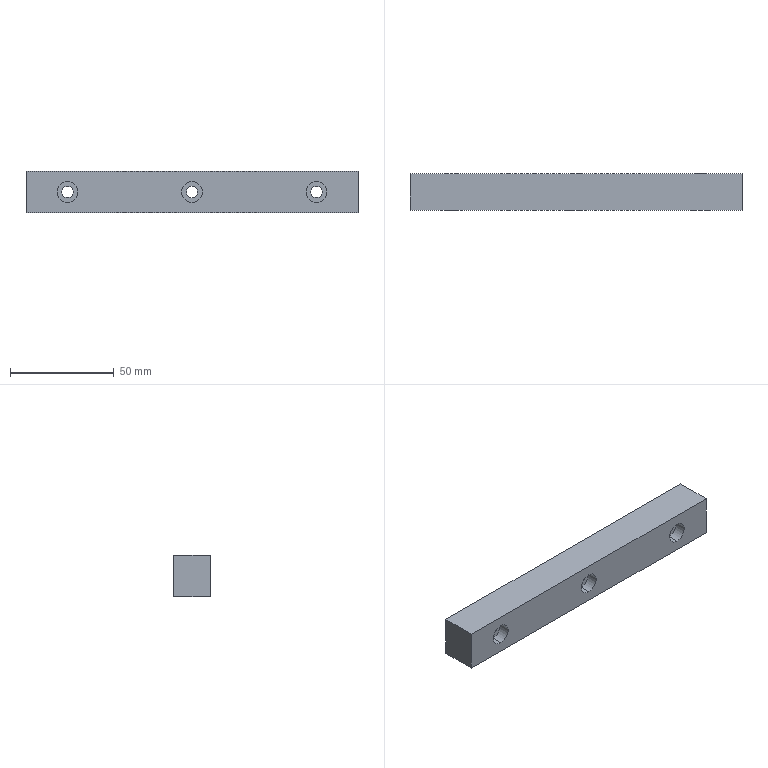Component | SolidWorks | GuideRailHIWINHGH20CA1R220-Z0-C-1 | 1 solid | 21 faces | box 160 x 17.5 x 20 mm | volume 53865 mm3 | cylinder 12 | plane 9 | commonest cylinder face diameters 5.5 x6 10 x6
build123d program:
from build123d import *

# Parameters (mm, degrees)
SKETCH1_W                                           = 160
SKETCH1_H                                           = 20
EXTRUDE1_DEPTH                                      = 17.5
CBORE_FOR_M5_HEX_SOCKET_HEAD_CAP_SCREW1_D           = 5.5
CBORE_FOR_M5_HEX_SOCKET_HEAD_CAP_SCREW1_CBORE_D     = 10
CBORE_FOR_M5_HEX_SOCKET_HEAD_CAP_SCREW1_CBORE_DEPTH = 5.4
LPATTERN1_COUNT                                     = 3
LPATTERN1_PITCH                                     = 60


with BuildPart() as part:
    # Sketch1 → Extrude1 (new body)
    with BuildSketch(Plane(origin=(0, 0, 0), x_dir=(1, 0, 0), z_dir=(0, 1, 0))):
        Rectangle(SKETCH1_W, SKETCH1_H)
    extrude(amount=EXTRUDE1_DEPTH)

    # CBORE for M5 Hex Socket Head Cap Screw1 (through all)
    with Locations(Plane(origin=(0, 17.5, 0), x_dir=(-1, 0, 0), z_dir=(0, 1, 0))):
        with Locations((-60, 0)):
            cbore_for_m5_hex_socket_head_cap_screw1 = CounterBoreHole(CBORE_FOR_M5_HEX_SOCKET_HEAD_CAP_SCREW1_D / 2, CBORE_FOR_M5_HEX_SOCKET_HEAD_CAP_SCREW1_CBORE_D / 2, CBORE_FOR_M5_HEX_SOCKET_HEAD_CAP_SCREW1_CBORE_DEPTH)

    # LPattern1: CBORE for M5 Hex Socket Head Cap Screw1 ×3
    with Locations(*[(-i * LPATTERN1_PITCH, 0, 0) for i in range(1, LPATTERN1_COUNT)]):
        add(cbore_for_m5_hex_socket_head_cap_screw1, mode=Mode.SUBTRACT)


solid = part.part

# Placed as in the assembly
solid = solid.moved(Location((-41.5, -10, -55), (180, 0, 0)))
STEP:
#1=COLOUR_RGB('',0.7922,0.8196,0.9333);
#2=FILL_AREA_STYLE_COLOUR('',#1);
#3=FILL_AREA_STYLE('',(#2));
#4=SURFACE_STYLE_FILL_AREA(#3);
#5=SURFACE_SIDE_STYLE('',(#4));
#6=SURFACE_STYLE_USAGE(.BOTH.,#5);
#7=PRESENTATION_STYLE_ASSIGNMENT((#6));
#8=CARTESIAN_POINT('',(0.7283,-0.3937,-2.274));
#9=VERTEX_POINT('',#8);
#10=CARTESIAN_POINT('',(0.7283,-0.3937,-2.057));
#11=VERTEX_POINT('',#10);
#12=CARTESIAN_POINT('',(0.7283,-0.3937,-2.165));
#13=DIRECTION('',(-0.,-1.,0.));
#14=DIRECTION('',(0.,0.,1.));
#15=AXIS2_PLACEMENT_3D('',#12,#13,#14);
#16=CIRCLE('',#15,0.1083);
#17=EDGE_CURVE('',#9,#11,#16,.T.);
#18=ORIENTED_EDGE('',*,*,#17,.F.);
#19=CARTESIAN_POINT('',(0.7283,-0.8701,-2.274));
#20=VERTEX_POINT('',#19);
#21=CARTESIAN_POINT('',(0.7283,-1.083,-2.274));
#22=DIRECTION('',(-0.,-1.,0.));
#23=VECTOR('',#22,39.37);
#24=LINE('',#21,#23);
#25=EDGE_CURVE('',#9,#20,#24,.T.);
#26=ORIENTED_EDGE('',*,*,#25,.T.);
#27=CARTESIAN_POINT('',(0.7283,-0.8701,-2.057));
#28=VERTEX_POINT('',#27);
#29=CARTESIAN_POINT('',(0.7283,-0.8701,-2.165));
#30=DIRECTION('',(-0.,-1.,0.));
#31=DIRECTION('',(0.,0.,1.));
#32=AXIS2_PLACEMENT_3D('',#29,#30,#31);
#33=CIRCLE('',#32,0.1083);
#34=EDGE_CURVE('',#20,#28,#33,.T.);
#35=ORIENTED_EDGE('',*,*,#34,.T.);
#36=CARTESIAN_POINT('',(0.7283,-1.083,-2.057));
#37=DIRECTION('',(-0.,-1.,0.));
#38=VECTOR('',#37,39.37);
#39=LINE('',#36,#38);
#40=EDGE_CURVE('',#11,#28,#39,.T.);
#41=ORIENTED_EDGE('',*,*,#40,.F.);
#42=EDGE_LOOP('',(#18,#26,#35,#41));
#43=FACE_OUTER_BOUND('',#42,.T.);
#44=CARTESIAN_POINT('',(0.7283,-1.083,-2.165));
#45=DIRECTION('',(-0.,-1.,0.));
#46=DIRECTION('',(0.,0.,1.));
#47=AXIS2_PLACEMENT_3D('',#44,#45,#46);
#48=CYLINDRICAL_SURFACE('',#47,0.1083);
#49=ADVANCED_FACE('',(#43),#48,.F.);
#50=CARTESIAN_POINT('',(0.7283,-0.8701,-2.362));
#51=VERTEX_POINT('',#50);
#52=CARTESIAN_POINT('',(0.7283,-0.8701,-1.969));
#53=VERTEX_POINT('',#52);
#54=CARTESIAN_POINT('',(0.7283,-0.8701,-2.165));
#55=DIRECTION('',(-0.,-1.,0.));
#56=DIRECTION('',(0.,0.,1.));
#57=AXIS2_PLACEMENT_3D('',#54,#55,#56);
#58=CIRCLE('',#57,0.1969);
#59=EDGE_CURVE('',#51,#53,#58,.T.);
#60=ORIENTED_EDGE('',*,*,#59,.F.);
#61=CARTESIAN_POINT('',(0.7283,-1.083,-2.362));
#62=VERTEX_POINT('',#61);
#63=CARTESIAN_POINT('',(0.7283,-1.083,-2.362));
#64=DIRECTION('',(-0.,-1.,0.));
#65=VECTOR('',#64,39.37);
#66=LINE('',#63,#65);
#67=EDGE_CURVE('',#51,#62,#66,.T.);
#68=ORIENTED_EDGE('',*,*,#67,.T.);
#69=CARTESIAN_POINT('',(0.7283,-1.083,-1.969));
#70=VERTEX_POINT('',#69);
#71=CARTESIAN_POINT('',(0.7283,-1.083,-2.165));
#72=DIRECTION('',(-0.,-1.,0.));
#73=DIRECTION('',(0.,0.,1.));
#74=AXIS2_PLACEMENT_3D('',#71,#72,#73);
#75=CIRCLE('',#74,0.1969);
#76=EDGE_CURVE('',#62,#70,#75,.T.);
#77=ORIENTED_EDGE('',*,*,#76,.T.);
#78=CARTESIAN_POINT('',(0.7283,-1.083,-1.969));
#79=DIRECTION('',(-0.,-1.,0.));
#80=VECTOR('',#79,39.37);
#81=LINE('',#78,#80);
#82=EDGE_CURVE('',#53,#70,#81,.T.);
#83=ORIENTED_EDGE('',*,*,#82,.F.);
#84=EDGE_LOOP('',(#60,#68,#77,#83));
#85=FACE_OUTER_BOUND('',#84,.T.);
#86=CARTESIAN_POINT('',(0.7283,-1.083,-2.165));
#87=DIRECTION('',(-0.,-1.,0.));
#88=DIRECTION('',(0.,0.,1.));
#89=AXIS2_PLACEMENT_3D('',#86,#87,#88);
#90=CYLINDRICAL_SURFACE('',#89,0.1969);
#91=ADVANCED_FACE('',(#85),#90,.F.);
#92=CARTESIAN_POINT('',(-1.634,-0.8701,-2.362));
#93=VERTEX_POINT('',#92);
#94=CARTESIAN_POINT('',(-1.634,-0.8701,-1.969));
#95=VERTEX_POINT('',#94);
#96=CARTESIAN_POINT('',(-1.634,-0.8701,-2.165));
#97=DIRECTION('',(-0.,-1.,0.));
#98=DIRECTION('',(0.,0.,1.));
#99=AXIS2_PLACEMENT_3D('',#96,#97,#98);
#100=CIRCLE('',#99,0.1969);
#101=EDGE_CURVE('',#93,#95,#100,.T.);
#102=ORIENTED_EDGE('',*,*,#101,.F.);
#103=CARTESIAN_POINT('',(-1.634,-1.083,-2.362));
#104=VERTEX_POINT('',#103);
#105=CARTESIAN_POINT('',(-1.634,-1.083,-2.362));
#106=DIRECTION('',(-0.,-1.,0.));
#107=VECTOR('',#106,39.37);
#108=LINE('',#105,#107);
#109=EDGE_CURVE('',#93,#104,#108,.T.);
#110=ORIENTED_EDGE('',*,*,#109,.T.);
#111=CARTESIAN_POINT('',(-1.634,-1.083,-1.969));
#112=VERTEX_POINT('',#111);
#113=CARTESIAN_POINT('',(-1.634,-1.083,-2.165));
#114=DIRECTION('',(-0.,-1.,0.));
#115=DIRECTION('',(0.,0.,1.));
#116=AXIS2_PLACEMENT_3D('',#113,#114,#115);
#117=CIRCLE('',#116,0.1969);
#118=EDGE_CURVE('',#104,#112,#117,.T.);
#119=ORIENTED_EDGE('',*,*,#118,.T.);
#120=CARTESIAN_POINT('',(-1.634,-1.083,-1.969));
#121=DIRECTION('',(-0.,-1.,0.));
#122=VECTOR('',#121,39.37);
#123=LINE('',#120,#122);
#124=EDGE_CURVE('',#95,#112,#123,.T.);
#125=ORIENTED_EDGE('',*,*,#124,.F.);
#126=EDGE_LOOP('',(#102,#110,#119,#125));
#127=FACE_OUTER_BOUND('',#126,.T.);
#128=CARTESIAN_POINT('',(-1.634,-1.083,-2.165));
#129=DIRECTION('',(-0.,-1.,0.));
#130=DIRECTION('',(0.,0.,1.));
#131=AXIS2_PLACEMENT_3D('',#128,#129,#130);
#132=CYLINDRICAL_SURFACE('',#131,0.1969);
#133=ADVANCED_FACE('',(#127),#132,.F.);
#134=CARTESIAN_POINT('',(-1.634,-0.3937,-2.274));
#135=VERTEX_POINT('',#134);
#136=CARTESIAN_POINT('',(-1.634,-0.3937,-2.057));
#137=VERTEX_POINT('',#136);
#138=CARTESIAN_POINT('',(-1.634,-0.3937,-2.165));
#139=DIRECTION('',(-0.,-1.,0.));
#140=DIRECTION('',(0.,0.,1.));
#141=AXIS2_PLACEMENT_3D('',#138,#139,#140);
#142=CIRCLE('',#141,0.1083);
#143=EDGE_CURVE('',#135,#137,#142,.T.);
#144=ORIENTED_EDGE('',*,*,#143,.F.);
#145=CARTESIAN_POINT('',(-1.634,-0.8701,-2.274));
#146=VERTEX_POINT('',#145);
#147=CARTESIAN_POINT('',(-1.634,-1.083,-2.274));
#148=DIRECTION('',(-0.,-1.,0.));
#149=VECTOR('',#148,39.37);
#150=LINE('',#147,#149);
#151=EDGE_CURVE('',#135,#146,#150,.T.);
#152=ORIENTED_EDGE('',*,*,#151,.T.);
#153=CARTESIAN_POINT('',(-1.634,-0.8701,-2.057));
#154=VERTEX_POINT('',#153);
#155=CARTESIAN_POINT('',(-1.634,-0.8701,-2.165));
#156=DIRECTION('',(-0.,-1.,0.));
#157=DIRECTION('',(0.,0.,1.));
#158=AXIS2_PLACEMENT_3D('',#155,#156,#157);
#159=CIRCLE('',#158,0.1083);
#160=EDGE_CURVE('',#146,#154,#159,.T.);
#161=ORIENTED_EDGE('',*,*,#160,.T.);
#162=CARTESIAN_POINT('',(-1.634,-1.083,-2.057));
#163=DIRECTION('',(-0.,-1.,0.));
#164=VECTOR('',#163,39.37);
#165=LINE('',#162,#164);
#166=EDGE_CURVE('',#137,#154,#165,.T.);
#167=ORIENTED_EDGE('',*,*,#166,.F.);
#168=EDGE_LOOP('',(#144,#152,#161,#167));
#169=FACE_OUTER_BOUND('',#168,.T.);
#170=CARTESIAN_POINT('',(-1.634,-1.083,-2.165));
#171=DIRECTION('',(-0.,-1.,0.));
#172=DIRECTION('',(0.,0.,1.));
#173=AXIS2_PLACEMENT_3D('',#170,#171,#172);
#174=CYLINDRICAL_SURFACE('',#173,0.1083);
#175=ADVANCED_FACE('',(#169),#174,.F.);
#176=CARTESIAN_POINT('',(-3.996,-0.8701,-2.362));
#177=VERTEX_POINT('',#176);
#178=CARTESIAN_POINT('',(-3.996,-0.8701,-1.969));
#179=VERTEX_POINT('',#178);
#180=CARTESIAN_POINT('',(-3.996,-0.8701,-2.165));
#181=DIRECTION('',(-0.,-1.,0.));
#182=DIRECTION('',(0.,0.,1.));
#183=AXIS2_PLACEMENT_3D('',#180,#181,#182);
#184=CIRCLE('',#183,0.1969);
#185=EDGE_CURVE('',#177,#179,#184,.T.);
#186=ORIENTED_EDGE('',*,*,#185,.F.);
#187=CARTESIAN_POINT('',(-3.996,-1.083,-2.362));
#188=VERTEX_POINT('',#187);
#189=CARTESIAN_POINT('',(-3.996,-1.083,-2.362));
#190=DIRECTION('',(-0.,-1.,0.));
#191=VECTOR('',#190,39.37);
#192=LINE('',#189,#191);
#193=EDGE_CURVE('',#177,#188,#192,.T.);
#194=ORIENTED_EDGE('',*,*,#193,.T.);
#195=CARTESIAN_POINT('',(-3.996,-1.083,-1.969));
#196=VERTEX_POINT('',#195);
#197=CARTESIAN_POINT('',(-3.996,-1.083,-2.165));
#198=DIRECTION('',(-0.,-1.,0.));
#199=DIRECTION('',(0.,0.,1.));
#200=AXIS2_PLACEMENT_3D('',#197,#198,#199);
#201=CIRCLE('',#200,0.1969);
#202=EDGE_CURVE('',#188,#196,#201,.T.);
#203=ORIENTED_EDGE('',*,*,#202,.T.);
#204=CARTESIAN_POINT('',(-3.996,-1.083,-1.969));
#205=DIRECTION('',(-0.,-1.,0.));
#206=VECTOR('',#205,39.37);
#207=LINE('',#204,#206);
#208=EDGE_CURVE('',#179,#196,#207,.T.);
#209=ORIENTED_EDGE('',*,*,#208,.F.);
#210=EDGE_LOOP('',(#186,#194,#203,#209));
#211=FACE_OUTER_BOUND('',#210,.T.);
#212=CARTESIAN_POINT('',(-3.996,-1.083,-2.165));
#213=DIRECTION('',(-0.,-1.,0.));
#214=DIRECTION('',(0.,0.,1.));
#215=AXIS2_PLACEMENT_3D('',#212,#213,#214);
#216=CYLINDRICAL_SURFACE('',#215,0.1969);
#217=ADVANCED_FACE('',(#211),#216,.F.);
#218=CARTESIAN_POINT('',(-3.996,-0.3937,-2.274));
#219=VERTEX_POINT('',#218);
#220=CARTESIAN_POINT('',(-3.996,-0.3937,-2.057));
#221=VERTEX_POINT('',#220);
#222=CARTESIAN_POINT('',(-3.996,-0.3937,-2.165));
#223=DIRECTION('',(-0.,-1.,0.));
#224=DIRECTION('',(0.,0.,1.));
#225=AXIS2_PLACEMENT_3D('',#222,#223,#224);
#226=CIRCLE('',#225,0.1083);
#227=EDGE_CURVE('',#219,#221,#226,.T.);
#228=ORIENTED_EDGE('',*,*,#227,.F.);
#229=CARTESIAN_POINT('',(-3.996,-0.8701,-2.274));
#230=VERTEX_POINT('',#229);
#231=CARTESIAN_POINT('',(-3.996,-1.083,-2.274));
#232=DIRECTION('',(-0.,-1.,0.));
#233=VECTOR('',#232,39.37);
#234=LINE('',#231,#233);
#235=EDGE_CURVE('',#219,#230,#234,.T.);
#236=ORIENTED_EDGE('',*,*,#235,.T.);
#237=CARTESIAN_POINT('',(-3.996,-0.8701,-2.057));
#238=VERTEX_POINT('',#237);
#239=CARTESIAN_POINT('',(-3.996,-0.8701,-2.165));
#240=DIRECTION('',(-0.,-1.,0.));
#241=DIRECTION('',(0.,0.,1.));
#242=AXIS2_PLACEMENT_3D('',#239,#240,#241);
#243=CIRCLE('',#242,0.1083);
#244=EDGE_CURVE('',#230,#238,#243,.T.);
#245=ORIENTED_EDGE('',*,*,#244,.T.);
#246=CARTESIAN_POINT('',(-3.996,-1.083,-2.057));
#247=DIRECTION('',(-0.,-1.,0.));
#248=VECTOR('',#247,39.37);
#249=LINE('',#246,#248);
#250=EDGE_CURVE('',#221,#238,#249,.T.);
#251=ORIENTED_EDGE('',*,*,#250,.F.);
#252=EDGE_LOOP('',(#228,#236,#245,#251));
#253=FACE_OUTER_BOUND('',#252,.T.);
#254=CARTESIAN_POINT('',(-3.996,-1.083,-2.165));
#255=DIRECTION('',(-0.,-1.,0.));
#256=DIRECTION('',(0.,0.,1.));
#257=AXIS2_PLACEMENT_3D('',#254,#255,#256);
#258=CYLINDRICAL_SURFACE('',#257,0.1083);
#259=ADVANCED_FACE('',(#253),#258,.F.);
#260=CARTESIAN_POINT('',(1.516,-0.3937,-2.559));
#261=VERTEX_POINT('',#260);
#262=CARTESIAN_POINT('',(1.516,-0.3937,-1.772));
#263=VERTEX_POINT('',#262);
#264=CARTESIAN_POINT('',(1.516,-0.3937,-2.559));
#265=DIRECTION('',(-0.,0.,1.));
#266=VECTOR('',#265,39.37);
#267=LINE('',#264,#266);
#268=EDGE_CURVE('',#261,#263,#267,.T.);
#269=ORIENTED_EDGE('',*,*,#268,.T.);
#270=CARTESIAN_POINT('',(1.516,-1.083,-1.772));
#271=VERTEX_POINT('',#270);
#272=CARTESIAN_POINT('',(1.516,-1.083,-1.772));
#273=DIRECTION('',(0.,1.,-0.));
#274=VECTOR('',#273,39.37);
#275=LINE('',#272,#274);
#276=EDGE_CURVE('',#271,#263,#275,.T.);
#277=ORIENTED_EDGE('',*,*,#276,.F.);
#278=CARTESIAN_POINT('',(1.516,-1.083,-2.559));
#279=VERTEX_POINT('',#278);
#280=CARTESIAN_POINT('',(1.516,-1.083,-2.559));
#281=DIRECTION('',(-0.,0.,1.));
#282=VECTOR('',#281,39.37);
#283=LINE('',#280,#282);
#284=EDGE_CURVE('',#279,#271,#283,.T.);
#285=ORIENTED_EDGE('',*,*,#284,.F.);
#286=CARTESIAN_POINT('',(1.516,-1.083,-2.559));
#287=DIRECTION('',(0.,1.,-0.));
#288=VECTOR('',#287,39.37);
#289=LINE('',#286,#288);
#290=EDGE_CURVE('',#279,#261,#289,.T.);
#291=ORIENTED_EDGE('',*,*,#290,.T.);
#292=EDGE_LOOP('',(#269,#277,#285,#291));
#293=FACE_OUTER_BOUND('',#292,.T.);
#294=CARTESIAN_POINT('',(1.516,-1.083,-2.559));
#295=DIRECTION('',(-1.,0.,-0.));
#296=DIRECTION('',(0.,-0.,-1.));
#297=AXIS2_PLACEMENT_3D('',#294,#295,#296);
#298=PLANE('',#297);
#299=ADVANCED_FACE('',(#293),#298,.F.);
#300=CARTESIAN_POINT('',(-4.783,-0.3937,-1.772));
#301=VERTEX_POINT('',#300);
#302=CARTESIAN_POINT('',(1.516,-0.3937,-1.772));
#303=DIRECTION('',(-1.,0.,-0.));
#304=VECTOR('',#303,39.37);
#305=LINE('',#302,#304);
#306=EDGE_CURVE('',#263,#301,#305,.T.);
#307=ORIENTED_EDGE('',*,*,#306,.T.);
#308=CARTESIAN_POINT('',(-4.783,-1.083,-1.772));
#309=VERTEX_POINT('',#308);
#310=CARTESIAN_POINT('',(-4.783,-1.083,-1.772));
#311=DIRECTION('',(0.,1.,-0.));
#312=VECTOR('',#311,39.37);
#313=LINE('',#310,#312);
#314=EDGE_CURVE('',#309,#301,#313,.T.);
#315=ORIENTED_EDGE('',*,*,#314,.F.);
#316=CARTESIAN_POINT('',(1.516,-1.083,-1.772));
#317=DIRECTION('',(-1.,0.,-0.));
#318=VECTOR('',#317,39.37);
#319=LINE('',#316,#318);
#320=EDGE_CURVE('',#271,#309,#319,.T.);
#321=ORIENTED_EDGE('',*,*,#320,.F.);
#322=ORIENTED_EDGE('',*,*,#276,.T.);
#323=EDGE_LOOP('',(#307,#315,#321,#322));
#324=FACE_OUTER_BOUND('',#323,.T.);
#325=CARTESIAN_POINT('',(1.516,-1.083,-1.772));
#326=DIRECTION('',(0.,-0.,-1.));
#327=DIRECTION('',(1.,-0.,0.));
#328=AXIS2_PLACEMENT_3D('',#325,#326,#327);
#329=PLANE('',#328);
#330=ADVANCED_FACE('',(#324),#329,.F.);
#331=CARTESIAN_POINT('',(-4.783,-0.3937,-2.559));
#332=VERTEX_POINT('',#331);
#333=CARTESIAN_POINT('',(-4.783,-0.3937,-2.559));
#334=DIRECTION('',(0.,-0.,-1.));
#335=VECTOR('',#334,39.37);
#336=LINE('',#333,#335);
#337=EDGE_CURVE('',#301,#332,#336,.T.);
#338=ORIENTED_EDGE('',*,*,#337,.T.);
#339=CARTESIAN_POINT('',(-4.783,-1.083,-2.559));
#340=VERTEX_POINT('',#339);
#341=CARTESIAN_POINT('',(-4.783,-1.083,-2.559));
#342=DIRECTION('',(0.,1.,-0.));
#343=VECTOR('',#342,39.37);
#344=LINE('',#341,#343);
#345=EDGE_CURVE('',#340,#332,#344,.T.);
#346=ORIENTED_EDGE('',*,*,#345,.F.);
#347=CARTESIAN_POINT('',(-4.783,-1.083,-2.559));
#348=DIRECTION('',(0.,-0.,-1.));
#349=VECTOR('',#348,39.37);
#350=LINE('',#347,#349);
#351=EDGE_CURVE('',#309,#340,#350,.T.);
#352=ORIENTED_EDGE('',*,*,#351,.F.);
#353=ORIENTED_EDGE('',*,*,#314,.T.);
#354=EDGE_LOOP('',(#338,#346,#352,#353));
#355=FACE_OUTER_BOUND('',#354,.T.);
#356=CARTESIAN_POINT('',(-4.783,-1.083,-2.559));
#357=DIRECTION('',(1.,-0.,0.));
#358=DIRECTION('',(-0.,0.,1.));
#359=AXIS2_PLACEMENT_3D('',#356,#357,#358);
#360=PLANE('',#359);
#361=ADVANCED_FACE('',(#355),#360,.F.);
#362=CARTESIAN_POINT('',(1.516,-0.3937,-2.559));
#363=DIRECTION('',(1.,-0.,0.));
#364=VECTOR('',#363,39.37);
#365=LINE('',#362,#364);
#366=EDGE_CURVE('',#332,#261,#365,.T.);
#367=ORIENTED_EDGE('',*,*,#366,.T.);
#368=ORIENTED_EDGE('',*,*,#290,.F.);
#369=CARTESIAN_POINT('',(1.516,-1.083,-2.559));
#370=DIRECTION('',(1.,-0.,0.));
#371=VECTOR('',#370,39.37);
#372=LINE('',#369,#371);
#373=EDGE_CURVE('',#340,#279,#372,.T.);
#374=ORIENTED_EDGE('',*,*,#373,.F.);
#375=ORIENTED_EDGE('',*,*,#345,.T.);
#376=EDGE_LOOP('',(#367,#368,#374,#375));
#377=FACE_OUTER_BOUND('',#376,.T.);
#378=CARTESIAN_POINT('',(1.516,-1.083,-2.559));
#379=DIRECTION('',(-0.,0.,1.));
#380=DIRECTION('',(-1.,0.,-0.));
#381=AXIS2_PLACEMENT_3D('',#378,#379,#380);
#382=PLANE('',#381);
#383=ADVANCED_FACE('',(#377),#382,.F.);
#384=CARTESIAN_POINT('',(-1.634,-1.083,-2.165));
#385=DIRECTION('',(-0.,-1.,0.));
#386=DIRECTION('',(0.,0.,1.));
#387=AXIS2_PLACEMENT_3D('',#384,#385,#386);
#388=CIRCLE('',#387,0.1969);
#389=EDGE_CURVE('',#112,#104,#388,.T.);
#390=ORIENTED_EDGE('',*,*,#389,.F.);
#391=ORIENTED_EDGE('',*,*,#118,.F.);
#392=EDGE_LOOP('',(#390,#391));
#393=FACE_BOUND('',#392,.T.);
#394=CARTESIAN_POINT('',(-3.996,-1.083,-2.165));
#395=DIRECTION('',(-0.,-1.,0.));
#396=DIRECTION('',(0.,0.,1.));
#397=AXIS2_PLACEMENT_3D('',#394,#395,#396);
#398=CIRCLE('',#397,0.1969);
#399=EDGE_CURVE('',#196,#188,#398,.T.);
#400=ORIENTED_EDGE('',*,*,#399,.F.);
#401=ORIENTED_EDGE('',*,*,#202,.F.);
#402=EDGE_LOOP('',(#400,#401));
#403=FACE_BOUND('',#402,.T.);
#404=ORIENTED_EDGE('',*,*,#284,.T.);
#405=ORIENTED_EDGE('',*,*,#320,.T.);
#406=ORIENTED_EDGE('',*,*,#351,.T.);
#407=ORIENTED_EDGE('',*,*,#373,.T.);
#408=EDGE_LOOP('',(#404,#405,#406,#407));
#409=FACE_OUTER_BOUND('',#408,.T.);
#410=CARTESIAN_POINT('',(0.7283,-1.083,-2.165));
#411=DIRECTION('',(-0.,-1.,0.));
#412=DIRECTION('',(0.,0.,1.));
#413=AXIS2_PLACEMENT_3D('',#410,#411,#412);
#414=CIRCLE('',#413,0.1969);
#415=EDGE_CURVE('',#70,#62,#414,.T.);
#416=ORIENTED_EDGE('',*,*,#415,.F.);
#417=ORIENTED_EDGE('',*,*,#76,.F.);
#418=EDGE_LOOP('',(#416,#417));
#419=FACE_BOUND('',#418,.T.);
#420=CARTESIAN_POINT('',(1.516,-1.083,-1.772));
#421=DIRECTION('',(-0.,-1.,0.));
#422=DIRECTION('',(-0.,0.,1.));
#423=AXIS2_PLACEMENT_3D('',#420,#421,#422);
#424=PLANE('',#423);
#425=ADVANCED_FACE('',(#393,#403,#409,#419),#424,.T.);
#426=CARTESIAN_POINT('',(-1.634,-0.3937,-2.165));
#427=DIRECTION('',(-0.,-1.,0.));
#428=DIRECTION('',(0.,0.,1.));
#429=AXIS2_PLACEMENT_3D('',#426,#427,#428);
#430=CIRCLE('',#429,0.1083);
#431=EDGE_CURVE('',#137,#135,#430,.T.);
#432=ORIENTED_EDGE('',*,*,#431,.T.);
#433=ORIENTED_EDGE('',*,*,#143,.T.);
#434=EDGE_LOOP('',(#432,#433));
#435=FACE_BOUND('',#434,.T.);
#436=CARTESIAN_POINT('',(-3.996,-0.3937,-2.165));
#437=DIRECTION('',(-0.,-1.,0.));
#438=DIRECTION('',(0.,0.,1.));
#439=AXIS2_PLACEMENT_3D('',#436,#437,#438);
#440=CIRCLE('',#439,0.1083);
#441=EDGE_CURVE('',#221,#219,#440,.T.);
#442=ORIENTED_EDGE('',*,*,#441,.T.);
#443=ORIENTED_EDGE('',*,*,#227,.T.);
#444=EDGE_LOOP('',(#442,#443));
#445=FACE_BOUND('',#444,.T.);
#446=ORIENTED_EDGE('',*,*,#268,.F.);
#447=ORIENTED_EDGE('',*,*,#366,.F.);
#448=ORIENTED_EDGE('',*,*,#337,.F.);
#449=ORIENTED_EDGE('',*,*,#306,.F.);
#450=EDGE_LOOP('',(#446,#447,#448,#449));
#451=FACE_OUTER_BOUND('',#450,.T.);
#452=CARTESIAN_POINT('',(0.7283,-0.3937,-2.165));
#453=DIRECTION('',(-0.,-1.,0.));
#454=DIRECTION('',(0.,0.,1.));
#455=AXIS2_PLACEMENT_3D('',#452,#453,#454);
#456=CIRCLE('',#455,0.1083);
#457=EDGE_CURVE('',#11,#9,#456,.T.);
#458=ORIENTED_EDGE('',*,*,#457,.T.);
#459=ORIENTED_EDGE('',*,*,#17,.T.);
#460=EDGE_LOOP('',(#458,#459));
#461=FACE_BOUND('',#460,.T.);
#462=CARTESIAN_POINT('',(1.516,-0.3937,-1.772));
#463=DIRECTION('',(-0.,-1.,0.));
#464=DIRECTION('',(-0.,0.,1.));
#465=AXIS2_PLACEMENT_3D('',#462,#463,#464);
#466=PLANE('',#465);
#467=ADVANCED_FACE('',(#435,#445,#451,#461),#466,.F.);
#468=ORIENTED_EDGE('',*,*,#235,.F.);
#469=ORIENTED_EDGE('',*,*,#441,.F.);
#470=ORIENTED_EDGE('',*,*,#250,.T.);
#471=CARTESIAN_POINT('',(-3.996,-0.8701,-2.165));
#472=DIRECTION('',(-0.,-1.,0.));
#473=DIRECTION('',(0.,0.,1.));
#474=AXIS2_PLACEMENT_3D('',#471,#472,#473);
#475=CIRCLE('',#474,0.1083);
#476=EDGE_CURVE('',#238,#230,#475,.T.);
#477=ORIENTED_EDGE('',*,*,#476,.T.);
#478=EDGE_LOOP('',(#468,#469,#470,#477));
#479=FACE_OUTER_BOUND('',#478,.T.);
#480=CARTESIAN_POINT('',(-3.996,-1.083,-2.165));
#481=DIRECTION('',(-0.,-1.,0.));
#482=DIRECTION('',(0.,0.,1.));
#483=AXIS2_PLACEMENT_3D('',#480,#481,#482);
#484=CYLINDRICAL_SURFACE('',#483,0.1083);
#485=ADVANCED_FACE('',(#479),#484,.F.);
#486=ORIENTED_EDGE('',*,*,#476,.F.);
#487=ORIENTED_EDGE('',*,*,#244,.F.);
#488=EDGE_LOOP('',(#486,#487));
#489=FACE_BOUND('',#488,.T.);
#490=CARTESIAN_POINT('',(-3.996,-0.8701,-2.165));
#491=DIRECTION('',(-0.,-1.,0.));
#492=DIRECTION('',(0.,0.,1.));
#493=AXIS2_PLACEMENT_3D('',#490,#491,#492);
#494=CIRCLE('',#493,0.1969);
#495=EDGE_CURVE('',#179,#177,#494,.T.);
#496=ORIENTED_EDGE('',*,*,#495,.T.);
#497=ORIENTED_EDGE('',*,*,#185,.T.);
#498=EDGE_LOOP('',(#496,#497));
#499=FACE_OUTER_BOUND('',#498,.T.);
#500=CARTESIAN_POINT('',(-4.104,-0.8701,-2.165));
#501=DIRECTION('',(0.,1.,-0.));
#502=DIRECTION('',(0.,-0.,-1.));
#503=AXIS2_PLACEMENT_3D('',#500,#501,#502);
#504=PLANE('',#503);
#505=ADVANCED_FACE('',(#489,#499),#504,.F.);
#506=ORIENTED_EDGE('',*,*,#193,.F.);
#507=ORIENTED_EDGE('',*,*,#495,.F.);
#508=ORIENTED_EDGE('',*,*,#208,.T.);
#509=ORIENTED_EDGE('',*,*,#399,.T.);
#510=EDGE_LOOP('',(#506,#507,#508,#509));
#511=FACE_OUTER_BOUND('',#510,.T.);
#512=CARTESIAN_POINT('',(-3.996,-1.083,-2.165));
#513=DIRECTION('',(-0.,-1.,0.));
#514=DIRECTION('',(0.,0.,1.));
#515=AXIS2_PLACEMENT_3D('',#512,#513,#514);
#516=CYLINDRICAL_SURFACE('',#515,0.1969);
#517=ADVANCED_FACE('',(#511),#516,.F.);
#518=ORIENTED_EDGE('',*,*,#151,.F.);
#519=ORIENTED_EDGE('',*,*,#431,.F.);
#520=ORIENTED_EDGE('',*,*,#166,.T.);
#521=CARTESIAN_POINT('',(-1.634,-0.8701,-2.165));
#522=DIRECTION('',(-0.,-1.,0.));
#523=DIRECTION('',(0.,0.,1.));
#524=AXIS2_PLACEMENT_3D('',#521,#522,#523);
#525=CIRCLE('',#524,0.1083);
#526=EDGE_CURVE('',#154,#146,#525,.T.);
#527=ORIENTED_EDGE('',*,*,#526,.T.);
#528=EDGE_LOOP('',(#518,#519,#520,#527));
#529=FACE_OUTER_BOUND('',#528,.T.);
#530=CARTESIAN_POINT('',(-1.634,-1.083,-2.165));
#531=DIRECTION('',(-0.,-1.,0.));
#532=DIRECTION('',(0.,0.,1.));
#533=AXIS2_PLACEMENT_3D('',#530,#531,#532);
#534=CYLINDRICAL_SURFACE('',#533,0.1083);
#535=ADVANCED_FACE('',(#529),#534,.F.);
#536=ORIENTED_EDGE('',*,*,#526,.F.);
#537=ORIENTED_EDGE('',*,*,#160,.F.);
#538=EDGE_LOOP('',(#536,#537));
#539=FACE_BOUND('',#538,.T.);
#540=CARTESIAN_POINT('',(-1.634,-0.8701,-2.165));
#541=DIRECTION('',(-0.,-1.,0.));
#542=DIRECTION('',(0.,0.,1.));
#543=AXIS2_PLACEMENT_3D('',#540,#541,#542);
#544=CIRCLE('',#543,0.1969);
#545=EDGE_CURVE('',#95,#93,#544,.T.);
#546=ORIENTED_EDGE('',*,*,#545,.T.);
#547=ORIENTED_EDGE('',*,*,#101,.T.);
#548=EDGE_LOOP('',(#546,#547));
#549=FACE_OUTER_BOUND('',#548,.T.);
#550=CARTESIAN_POINT('',(-1.742,-0.8701,-2.165));
#551=DIRECTION('',(0.,1.,-0.));
#552=DIRECTION('',(0.,-0.,-1.));
#553=AXIS2_PLACEMENT_3D('',#550,#551,#552);
#554=PLANE('',#553);
#555=ADVANCED_FACE('',(#539,#549),#554,.F.);
#556=ORIENTED_EDGE('',*,*,#109,.F.);
#557=ORIENTED_EDGE('',*,*,#545,.F.);
#558=ORIENTED_EDGE('',*,*,#124,.T.);
#559=ORIENTED_EDGE('',*,*,#389,.T.);
#560=EDGE_LOOP('',(#556,#557,#558,#559));
#561=FACE_OUTER_BOUND('',#560,.T.);
#562=CARTESIAN_POINT('',(-1.634,-1.083,-2.165));
#563=DIRECTION('',(-0.,-1.,0.));
#564=DIRECTION('',(0.,0.,1.));
#565=AXIS2_PLACEMENT_3D('',#562,#563,#564);
#566=CYLINDRICAL_SURFACE('',#565,0.1969);
#567=ADVANCED_FACE('',(#561),#566,.F.);
#568=ORIENTED_EDGE('',*,*,#67,.F.);
#569=CARTESIAN_POINT('',(0.7283,-0.8701,-2.165));
#570=DIRECTION('',(-0.,-1.,0.));
#571=DIRECTION('',(0.,0.,1.));
#572=AXIS2_PLACEMENT_3D('',#569,#570,#571);
#573=CIRCLE('',#572,0.1969);
#574=EDGE_CURVE('',#53,#51,#573,.T.);
#575=ORIENTED_EDGE('',*,*,#574,.F.);
#576=ORIENTED_EDGE('',*,*,#82,.T.);
#577=ORIENTED_EDGE('',*,*,#415,.T.);
#578=EDGE_LOOP('',(#568,#575,#576,#577));
#579=FACE_OUTER_BOUND('',#578,.T.);
#580=CARTESIAN_POINT('',(0.7283,-1.083,-2.165));
#581=DIRECTION('',(-0.,-1.,0.));
#582=DIRECTION('',(0.,0.,1.));
#583=AXIS2_PLACEMENT_3D('',#580,#581,#582);
#584=CYLINDRICAL_SURFACE('',#583,0.1969);
#585=ADVANCED_FACE('',(#579),#584,.F.);
#586=CARTESIAN_POINT('',(0.7283,-0.8701,-2.165));
#587=DIRECTION('',(-0.,-1.,0.));
#588=DIRECTION('',(0.,0.,1.));
#589=AXIS2_PLACEMENT_3D('',#586,#587,#588);
#590=CIRCLE('',#589,0.1083);
#591=EDGE_CURVE('',#28,#20,#590,.T.);
#592=ORIENTED_EDGE('',*,*,#591,.F.);
#593=ORIENTED_EDGE('',*,*,#34,.F.);
#594=EDGE_LOOP('',(#592,#593));
#595=FACE_BOUND('',#594,.T.);
#596=ORIENTED_EDGE('',*,*,#574,.T.);
#597=ORIENTED_EDGE('',*,*,#59,.T.);
#598=EDGE_LOOP('',(#596,#597));
#599=FACE_OUTER_BOUND('',#598,.T.);
#600=CARTESIAN_POINT('',(0.6201,-0.8701,-2.165));
#601=DIRECTION('',(0.,1.,-0.));
#602=DIRECTION('',(0.,-0.,-1.));
#603=AXIS2_PLACEMENT_3D('',#600,#601,#602);
#604=PLANE('',#603);
#605=ADVANCED_FACE('',(#595,#599),#604,.F.);
#606=ORIENTED_EDGE('',*,*,#25,.F.);
#607=ORIENTED_EDGE('',*,*,#457,.F.);
#608=ORIENTED_EDGE('',*,*,#40,.T.);
#609=ORIENTED_EDGE('',*,*,#591,.T.);
#610=EDGE_LOOP('',(#606,#607,#608,#609));
#611=FACE_OUTER_BOUND('',#610,.T.);
#612=CARTESIAN_POINT('',(0.7283,-1.083,-2.165));
#613=DIRECTION('',(-0.,-1.,0.));
#614=DIRECTION('',(0.,0.,1.));
#615=AXIS2_PLACEMENT_3D('',#612,#613,#614);
#616=CYLINDRICAL_SURFACE('',#615,0.1083);
#617=ADVANCED_FACE('',(#611),#616,.F.);
#618=CLOSED_SHELL('',(#49,#91,#133,#175,#217,#259,#299,#330,#361,#383,#425,#467,#485,#505,#517,#535,#555,#567,#585,#605,#617));
#619=MANIFOLD_SOLID_BREP('',#618);
#620=STYLED_ITEM('',(#7),#619);
#621=PRESENTATION_LAYER_ASSIGNMENT('','',(#620));
#622=CARTESIAN_POINT('',(0.,0.,0.));
#623=DIRECTION('',(0.,0.,1.));
#624=DIRECTION('',(1.,0.,0.));
#625=AXIS2_PLACEMENT_3D('',#622,#623,#624);
#626=(LENGTH_UNIT()NAMED_UNIT(*)SI_UNIT($,.METRE.));
#627=LENGTH_MEASURE_WITH_UNIT(LENGTH_MEASURE(0.0254),#626);
#628=DIMENSIONAL_EXPONENTS(1.,0.,0.,0.,0.,0.,0.);
#629=(CONVERSION_BASED_UNIT('',#627)LENGTH_UNIT()NAMED_UNIT(#628));
#630=UNCERTAINTY_MEASURE_WITH_UNIT(LENGTH_MEASURE(0.00001),#629,'','');
#631=(NAMED_UNIT(*)PLANE_ANGLE_UNIT()SI_UNIT($,.RADIAN.));
#632=(NAMED_UNIT(*)SI_UNIT($,.STERADIAN.)SOLID_ANGLE_UNIT());
#633=(GEOMETRIC_REPRESENTATION_CONTEXT(3)GLOBAL_UNCERTAINTY_ASSIGNED_CONTEXT((#630))GLOBAL_UNIT_ASSIGNED_CONTEXT((#629,#631,#632))REPRESENTATION_CONTEXT('',''));
#634=ADVANCED_BREP_SHAPE_REPRESENTATION('',(#619,#625),#633);
#635=(LENGTH_UNIT()NAMED_UNIT(*)SI_UNIT($,.METRE.));
#636=LENGTH_MEASURE_WITH_UNIT(LENGTH_MEASURE(0.0254),#635);
#637=DIMENSIONAL_EXPONENTS(1.,0.,0.,0.,0.,0.,0.);
#638=(CONVERSION_BASED_UNIT('',#636)LENGTH_UNIT()NAMED_UNIT(#637));
#639=UNCERTAINTY_MEASURE_WITH_UNIT(LENGTH_MEASURE(0.00001),#638,'','');
#640=(NAMED_UNIT(*)PLANE_ANGLE_UNIT()SI_UNIT($,.RADIAN.));
#641=(NAMED_UNIT(*)SI_UNIT($,.STERADIAN.)SOLID_ANGLE_UNIT());
#642=(GEOMETRIC_REPRESENTATION_CONTEXT(3)GLOBAL_UNCERTAINTY_ASSIGNED_CONTEXT((#639))GLOBAL_UNIT_ASSIGNED_CONTEXT((#638,#640,#641))REPRESENTATION_CONTEXT('',''));
#643=MECHANICAL_DESIGN_GEOMETRIC_PRESENTATION_REPRESENTATION('',(#620),#642);